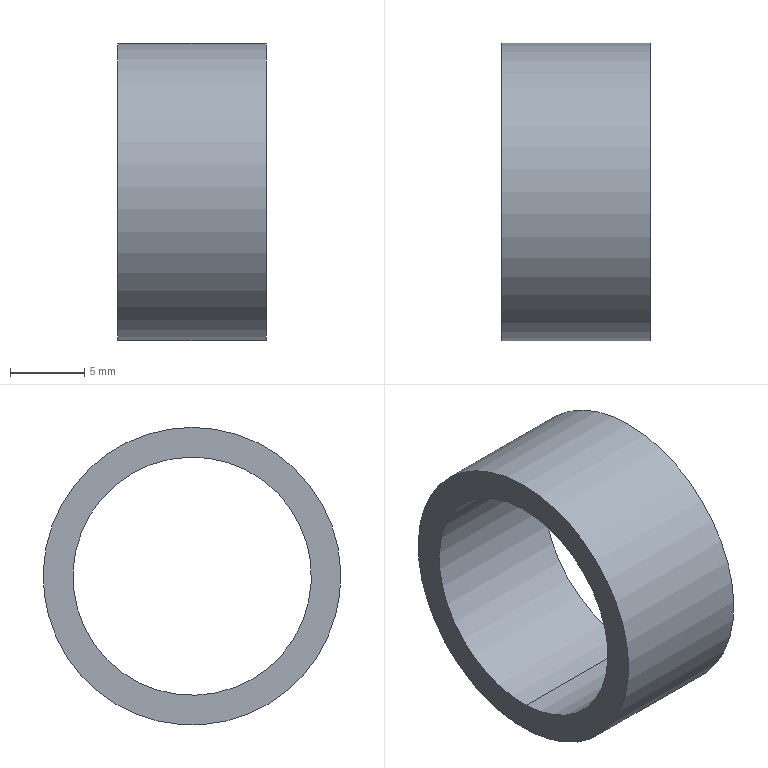Component | NX | BUSHING_2 | 1 solid | 5 faces | box 10 x 20 x 20 mm | volume 1127 mm3 | cylinder 3 | plane 2 | commonest cylinder face diameters 16 x2 20 x1
STEP:
#1=CARTESIAN_POINT('',(0.,0.,0.));
#2=DIRECTION('',(0.,0.,1.));
#3=DIRECTION('',(1.,0.,0.));
#4=AXIS2_PLACEMENT_3D('',#1,#2,#3);
#5=CARTESIAN_POINT('',(35.,80.231,-12.003));
#6=VERTEX_POINT('',#5);
#7=CARTESIAN_POINT('',(35.,79.744,-27.996));
#8=VERTEX_POINT('',#7);
#9=CARTESIAN_POINT('',(35.,80.,-20.));
#10=DIRECTION('',(-1.,0.,0.));
#11=DIRECTION('',(0.,0.,1.));
#12=AXIS2_PLACEMENT_3D('',#9,#10,#11);
#13=CIRCLE('',#12,8.);
#14=CARTESIAN_POINT('',(35.,80.,-20.));
#15=DIRECTION('',(-1.,0.,0.));
#16=DIRECTION('',(0.,0.,1.));
#17=AXIS2_PLACEMENT_3D('',#14,#15,#16);
#18=CYLINDRICAL_SURFACE('',#17,8.);
#19=CARTESIAN_POINT('',(0.,0.));
#20=DIRECTION('',(1.,0.));
#21=VECTOR('',#20,1.);
#22=LINE('',#19,#21);
#23=(GEOMETRIC_REPRESENTATION_CONTEXT(2)PARAMETRIC_REPRESENTATION_CONTEXT()REPRESENTATION_CONTEXT('',''));
#24=DEFINITIONAL_REPRESENTATION('',(#22),#23);
#25=PCURVE('',#18,#24);
#26=CARTESIAN_POINT('',(35.,80.,-20.));
#27=DIRECTION('',(-1.,0.,0.));
#28=DIRECTION('',(0.,0.,1.));
#29=AXIS2_PLACEMENT_3D('',#26,#27,#28);
#30=PLANE('',#29);
#31=CARTESIAN_POINT('',(0.,0.));
#32=DIRECTION('',(1.,0.));
#33=AXIS2_PLACEMENT_2D('',#31,#32);
#34=CIRCLE('',#33,8.);
#35=(GEOMETRIC_REPRESENTATION_CONTEXT(2)PARAMETRIC_REPRESENTATION_CONTEXT()REPRESENTATION_CONTEXT('',''));
#36=DEFINITIONAL_REPRESENTATION('',(#34),#35);
#37=PCURVE('',#30,#36);
#38=SURFACE_CURVE('',#13,(#25,#37),.PCURVE_S1.);
#39=EDGE_CURVE('',#6,#8,#38,.T.);
#40=ORIENTED_EDGE('',*,*,#39,.T.);
#41=CARTESIAN_POINT('',(25.,79.744,-27.996));
#42=VERTEX_POINT('',#41);
#43=CARTESIAN_POINT('',(30.,79.744,-27.996));
#44=DIRECTION('',(-1.,0.,0.));
#45=VECTOR('',#44,1.);
#46=LINE('',#43,#45);
#47=CARTESIAN_POINT('',(3.174,5.));
#48=DIRECTION('',(0.,1.));
#49=VECTOR('',#48,1.);
#50=LINE('',#47,#49);
#51=(GEOMETRIC_REPRESENTATION_CONTEXT(2)PARAMETRIC_REPRESENTATION_CONTEXT()REPRESENTATION_CONTEXT('',''));
#52=DEFINITIONAL_REPRESENTATION('',(#50),#51);
#53=PCURVE('',#18,#52);
#54=CARTESIAN_POINT('',(35.,79.975,-19.999));
#55=DIRECTION('',(-1.,0.,0.));
#56=DIRECTION('',(0.,-0.9995,0.03066));
#57=AXIS2_PLACEMENT_3D('',#54,#55,#56);
#58=CYLINDRICAL_SURFACE('',#57,8.);
#59=CARTESIAN_POINT('',(4.711,5.));
#60=DIRECTION('',(0.,1.));
#61=VECTOR('',#60,1.);
#62=LINE('',#59,#61);
#63=(GEOMETRIC_REPRESENTATION_CONTEXT(2)PARAMETRIC_REPRESENTATION_CONTEXT()REPRESENTATION_CONTEXT('',''));
#64=DEFINITIONAL_REPRESENTATION('',(#62),#63);
#65=PCURVE('',#58,#64);
#66=SURFACE_CURVE('',#46,(#53,#65),.PCURVE_S1.);
#67=EDGE_CURVE('',#8,#42,#66,.T.);
#68=ORIENTED_EDGE('',*,*,#67,.T.);
#69=CARTESIAN_POINT('',(25.,80.231,-12.003));
#70=VERTEX_POINT('',#69);
#71=CARTESIAN_POINT('',(25.,80.,-20.));
#72=DIRECTION('',(-1.,0.,0.));
#73=DIRECTION('',(0.,0.,1.));
#74=AXIS2_PLACEMENT_3D('',#71,#72,#73);
#75=CIRCLE('',#74,8.);
#76=CARTESIAN_POINT('',(0.,10.));
#77=DIRECTION('',(1.,0.));
#78=VECTOR('',#77,1.);
#79=LINE('',#76,#78);
#80=(GEOMETRIC_REPRESENTATION_CONTEXT(2)PARAMETRIC_REPRESENTATION_CONTEXT()REPRESENTATION_CONTEXT('',''));
#81=DEFINITIONAL_REPRESENTATION('',(#79),#80);
#82=PCURVE('',#18,#81);
#83=CARTESIAN_POINT('',(25.,80.,-20.));
#84=DIRECTION('',(-1.,0.,0.));
#85=DIRECTION('',(0.,0.,1.));
#86=AXIS2_PLACEMENT_3D('',#83,#84,#85);
#87=PLANE('',#86);
#88=CARTESIAN_POINT('',(0.,0.));
#89=DIRECTION('',(1.,0.));
#90=AXIS2_PLACEMENT_2D('',#88,#89);
#91=CIRCLE('',#90,8.);
#92=(GEOMETRIC_REPRESENTATION_CONTEXT(2)PARAMETRIC_REPRESENTATION_CONTEXT()REPRESENTATION_CONTEXT('',''));
#93=DEFINITIONAL_REPRESENTATION('',(#91),#92);
#94=PCURVE('',#87,#93);
#95=SURFACE_CURVE('',#75,(#82,#94),.PCURVE_S1.);
#96=EDGE_CURVE('',#70,#42,#95,.T.);
#97=ORIENTED_EDGE('',*,*,#96,.F.);
#98=CARTESIAN_POINT('',(30.,80.231,-12.003));
#99=DIRECTION('',(1.,0.,0.));
#100=VECTOR('',#99,1.);
#101=LINE('',#98,#100);
#102=CARTESIAN_POINT('',(0.02886,5.));
#103=DIRECTION('',(0.,-1.));
#104=VECTOR('',#103,1.);
#105=LINE('',#102,#104);
#106=(GEOMETRIC_REPRESENTATION_CONTEXT(2)PARAMETRIC_REPRESENTATION_CONTEXT()REPRESENTATION_CONTEXT('',''));
#107=DEFINITIONAL_REPRESENTATION('',(#105),#106);
#108=PCURVE('',#18,#107);
#109=CARTESIAN_POINT('',(7.855,5.));
#110=DIRECTION('',(0.,-1.));
#111=VECTOR('',#110,1.);
#112=LINE('',#109,#111);
#113=(GEOMETRIC_REPRESENTATION_CONTEXT(2)PARAMETRIC_REPRESENTATION_CONTEXT()REPRESENTATION_CONTEXT('',''));
#114=DEFINITIONAL_REPRESENTATION('',(#112),#113);
#115=PCURVE('',#58,#114);
#116=SURFACE_CURVE('',#101,(#108,#115),.PCURVE_S1.);
#117=EDGE_CURVE('',#70,#6,#116,.T.);
#118=ORIENTED_EDGE('',*,*,#117,.T.);
#119=EDGE_LOOP('',(#40,#68,#97,#118));
#120=FACE_BOUND('',#119,.F.);
#121=ADVANCED_FACE('',(#120),#18,.F.);
#122=CARTESIAN_POINT('',(35.,80.,-10.));
#123=VERTEX_POINT('',#122);
#124=CARTESIAN_POINT('',(35.,80.,-20.));
#125=DIRECTION('',(-1.,0.,0.));
#126=DIRECTION('',(0.,0.,1.));
#127=AXIS2_PLACEMENT_3D('',#124,#125,#126);
#128=CIRCLE('',#127,10.);
#129=CARTESIAN_POINT('',(0.,0.));
#130=DIRECTION('',(1.,0.));
#131=AXIS2_PLACEMENT_2D('',#129,#130);
#132=CIRCLE('',#131,10.);
#133=(GEOMETRIC_REPRESENTATION_CONTEXT(2)PARAMETRIC_REPRESENTATION_CONTEXT()REPRESENTATION_CONTEXT('',''));
#134=DEFINITIONAL_REPRESENTATION('',(#132),#133);
#135=PCURVE('',#30,#134);
#136=CARTESIAN_POINT('',(35.,80.,-20.));
#137=DIRECTION('',(-1.,0.,0.));
#138=DIRECTION('',(0.,0.,1.));
#139=AXIS2_PLACEMENT_3D('',#136,#137,#138);
#140=CYLINDRICAL_SURFACE('',#139,10.);
#141=CARTESIAN_POINT('',(0.,0.));
#142=DIRECTION('',(1.,0.));
#143=VECTOR('',#142,1.);
#144=LINE('',#141,#143);
#145=(GEOMETRIC_REPRESENTATION_CONTEXT(2)PARAMETRIC_REPRESENTATION_CONTEXT()REPRESENTATION_CONTEXT('',''));
#146=DEFINITIONAL_REPRESENTATION('',(#144),#145);
#147=PCURVE('',#140,#146);
#148=SURFACE_CURVE('',#128,(#135,#147),.PCURVE_S1.);
#149=EDGE_CURVE('',#123,#123,#148,.T.);
#150=ORIENTED_EDGE('',*,*,#149,.F.);
#151=EDGE_LOOP('',(#150));
#152=FACE_BOUND('',#151,.T.);
#153=ORIENTED_EDGE('',*,*,#39,.T.);
#154=CARTESIAN_POINT('',(35.,79.975,-19.999));
#155=DIRECTION('',(-1.,0.,0.));
#156=DIRECTION('',(0.,-0.0004954,-1.));
#157=AXIS2_PLACEMENT_3D('',#154,#155,#156);
#158=CIRCLE('',#157,8.);
#159=CARTESIAN_POINT('',(0.0007532,-0.02476));
#160=DIRECTION('',(-1.,-0.0004954));
#161=AXIS2_PLACEMENT_2D('',#159,#160);
#162=CIRCLE('',#161,8.);
#163=(GEOMETRIC_REPRESENTATION_CONTEXT(2)PARAMETRIC_REPRESENTATION_CONTEXT()REPRESENTATION_CONTEXT('',''));
#164=DEFINITIONAL_REPRESENTATION('',(#162),#163);
#165=PCURVE('',#30,#164);
#166=CARTESIAN_POINT('',(4.682,0.));
#167=DIRECTION('',(1.,0.));
#168=VECTOR('',#167,1.);
#169=LINE('',#166,#168);
#170=(GEOMETRIC_REPRESENTATION_CONTEXT(2)PARAMETRIC_REPRESENTATION_CONTEXT()REPRESENTATION_CONTEXT('',''));
#171=DEFINITIONAL_REPRESENTATION('',(#169),#170);
#172=PCURVE('',#58,#171);
#173=SURFACE_CURVE('',#158,(#165,#172),.PCURVE_S1.);
#174=EDGE_CURVE('',#8,#6,#173,.T.);
#175=ORIENTED_EDGE('',*,*,#174,.T.);
#176=EDGE_LOOP('',(#153,#175));
#177=FACE_BOUND('',#176,.T.);
#178=ADVANCED_FACE('',(#152,#177),#30,.F.);
#179=ORIENTED_EDGE('',*,*,#149,.T.);
#180=CARTESIAN_POINT('',(25.,80.,-10.));
#181=VERTEX_POINT('',#180);
#182=CARTESIAN_POINT('',(35.,80.,-10.));
#183=CARTESIAN_POINT('',(25.,80.,-10.));
#184=B_SPLINE_CURVE_WITH_KNOTS('',1,(#182,#183),.UNSPECIFIED.,.F.,.F.,(2,2),(0.,10.),.PIECEWISE_BEZIER_KNOTS.);
#185=CARTESIAN_POINT('',(6.283,0.));
#186=DIRECTION('',(0.,1.));
#187=VECTOR('',#186,1.);
#188=LINE('',#185,#187);
#189=(GEOMETRIC_REPRESENTATION_CONTEXT(2)PARAMETRIC_REPRESENTATION_CONTEXT()REPRESENTATION_CONTEXT('',''));
#190=DEFINITIONAL_REPRESENTATION('',(#188),#189);
#191=PCURVE('',#140,#190);
#192=CARTESIAN_POINT('',(0.,0.));
#193=DIRECTION('',(0.,1.));
#194=VECTOR('',#193,1.);
#195=LINE('',#192,#194);
#196=(GEOMETRIC_REPRESENTATION_CONTEXT(2)PARAMETRIC_REPRESENTATION_CONTEXT()REPRESENTATION_CONTEXT('',''));
#197=DEFINITIONAL_REPRESENTATION('',(#195),#196);
#198=PCURVE('',#140,#197);
#199=SEAM_CURVE('',#184,(#191,#198),.PCURVE_S1.);
#200=EDGE_CURVE('',#123,#181,#199,.T.);
#201=ORIENTED_EDGE('',*,*,#200,.T.);
#202=CARTESIAN_POINT('',(25.,80.,-20.));
#203=DIRECTION('',(-1.,0.,0.));
#204=DIRECTION('',(0.,0.,1.));
#205=AXIS2_PLACEMENT_3D('',#202,#203,#204);
#206=CIRCLE('',#205,10.);
#207=CARTESIAN_POINT('',(0.,10.));
#208=DIRECTION('',(1.,0.));
#209=VECTOR('',#208,1.);
#210=LINE('',#207,#209);
#211=(GEOMETRIC_REPRESENTATION_CONTEXT(2)PARAMETRIC_REPRESENTATION_CONTEXT()REPRESENTATION_CONTEXT('',''));
#212=DEFINITIONAL_REPRESENTATION('',(#210),#211);
#213=PCURVE('',#140,#212);
#214=CARTESIAN_POINT('',(0.,0.));
#215=DIRECTION('',(1.,0.));
#216=AXIS2_PLACEMENT_2D('',#214,#215);
#217=CIRCLE('',#216,10.);
#218=(GEOMETRIC_REPRESENTATION_CONTEXT(2)PARAMETRIC_REPRESENTATION_CONTEXT()REPRESENTATION_CONTEXT('',''));
#219=DEFINITIONAL_REPRESENTATION('',(#217),#218);
#220=PCURVE('',#87,#219);
#221=SURFACE_CURVE('',#206,(#213,#220),.PCURVE_S1.);
#222=EDGE_CURVE('',#181,#181,#221,.T.);
#223=ORIENTED_EDGE('',*,*,#222,.F.);
#224=ORIENTED_EDGE('',*,*,#200,.F.);
#225=EDGE_LOOP('',(#179,#201,#223,#224));
#226=FACE_BOUND('',#225,.T.);
#227=ADVANCED_FACE('',(#226),#140,.T.);
#228=ORIENTED_EDGE('',*,*,#222,.T.);
#229=EDGE_LOOP('',(#228));
#230=FACE_BOUND('',#229,.T.);
#231=CARTESIAN_POINT('',(25.,79.975,-19.999));
#232=DIRECTION('',(-1.,0.,0.));
#233=DIRECTION('',(0.,0.9995,-0.03066));
#234=AXIS2_PLACEMENT_3D('',#231,#232,#233);
#235=CIRCLE('',#234,8.);
#236=CARTESIAN_POINT('',(0.0007532,-0.02476));
#237=DIRECTION('',(-0.03066,0.9995));
#238=AXIS2_PLACEMENT_2D('',#236,#237);
#239=CIRCLE('',#238,8.);
#240=(GEOMETRIC_REPRESENTATION_CONTEXT(2)PARAMETRIC_REPRESENTATION_CONTEXT()REPRESENTATION_CONTEXT('',''));
#241=DEFINITIONAL_REPRESENTATION('',(#239),#240);
#242=PCURVE('',#87,#241);
#243=CARTESIAN_POINT('',(3.142,10.));
#244=DIRECTION('',(1.,0.));
#245=VECTOR('',#244,1.);
#246=LINE('',#243,#245);
#247=(GEOMETRIC_REPRESENTATION_CONTEXT(2)PARAMETRIC_REPRESENTATION_CONTEXT()REPRESENTATION_CONTEXT('',''));
#248=DEFINITIONAL_REPRESENTATION('',(#246),#247);
#249=PCURVE('',#58,#248);
#250=SURFACE_CURVE('',#235,(#242,#249),.PCURVE_S1.);
#251=EDGE_CURVE('',#42,#70,#250,.T.);
#252=ORIENTED_EDGE('',*,*,#251,.F.);
#253=ORIENTED_EDGE('',*,*,#96,.F.);
#254=EDGE_LOOP('',(#252,#253));
#255=FACE_BOUND('',#254,.T.);
#256=ADVANCED_FACE('',(#230,#255),#87,.T.);
#257=ORIENTED_EDGE('',*,*,#251,.F.);
#258=ORIENTED_EDGE('',*,*,#67,.F.);
#259=ORIENTED_EDGE('',*,*,#174,.T.);
#260=ORIENTED_EDGE('',*,*,#117,.F.);
#261=EDGE_LOOP('',(#257,#258,#259,#260));
#262=FACE_BOUND('',#261,.F.);
#263=ADVANCED_FACE('',(#262),#58,.F.);
#264=CLOSED_SHELL('',(#121,#178,#227,#256,#263));
#265=MANIFOLD_SOLID_BREP('',#264);
#266=(LENGTH_UNIT()NAMED_UNIT(*)SI_UNIT(.MILLI.,.METRE.));
#267=UNCERTAINTY_MEASURE_WITH_UNIT(LENGTH_MEASURE(0.000002),#266,'','');
#268=(NAMED_UNIT(*)PLANE_ANGLE_UNIT()SI_UNIT($,.RADIAN.));
#269=(NAMED_UNIT(*)SI_UNIT($,.STERADIAN.)SOLID_ANGLE_UNIT());
#270=(GEOMETRIC_REPRESENTATION_CONTEXT(3)GLOBAL_UNCERTAINTY_ASSIGNED_CONTEXT((#267))GLOBAL_UNIT_ASSIGNED_CONTEXT((#266,#268,#269))REPRESENTATION_CONTEXT('',''));
#271=ADVANCED_BREP_SHAPE_REPRESENTATION('',(#4,#265),#270);